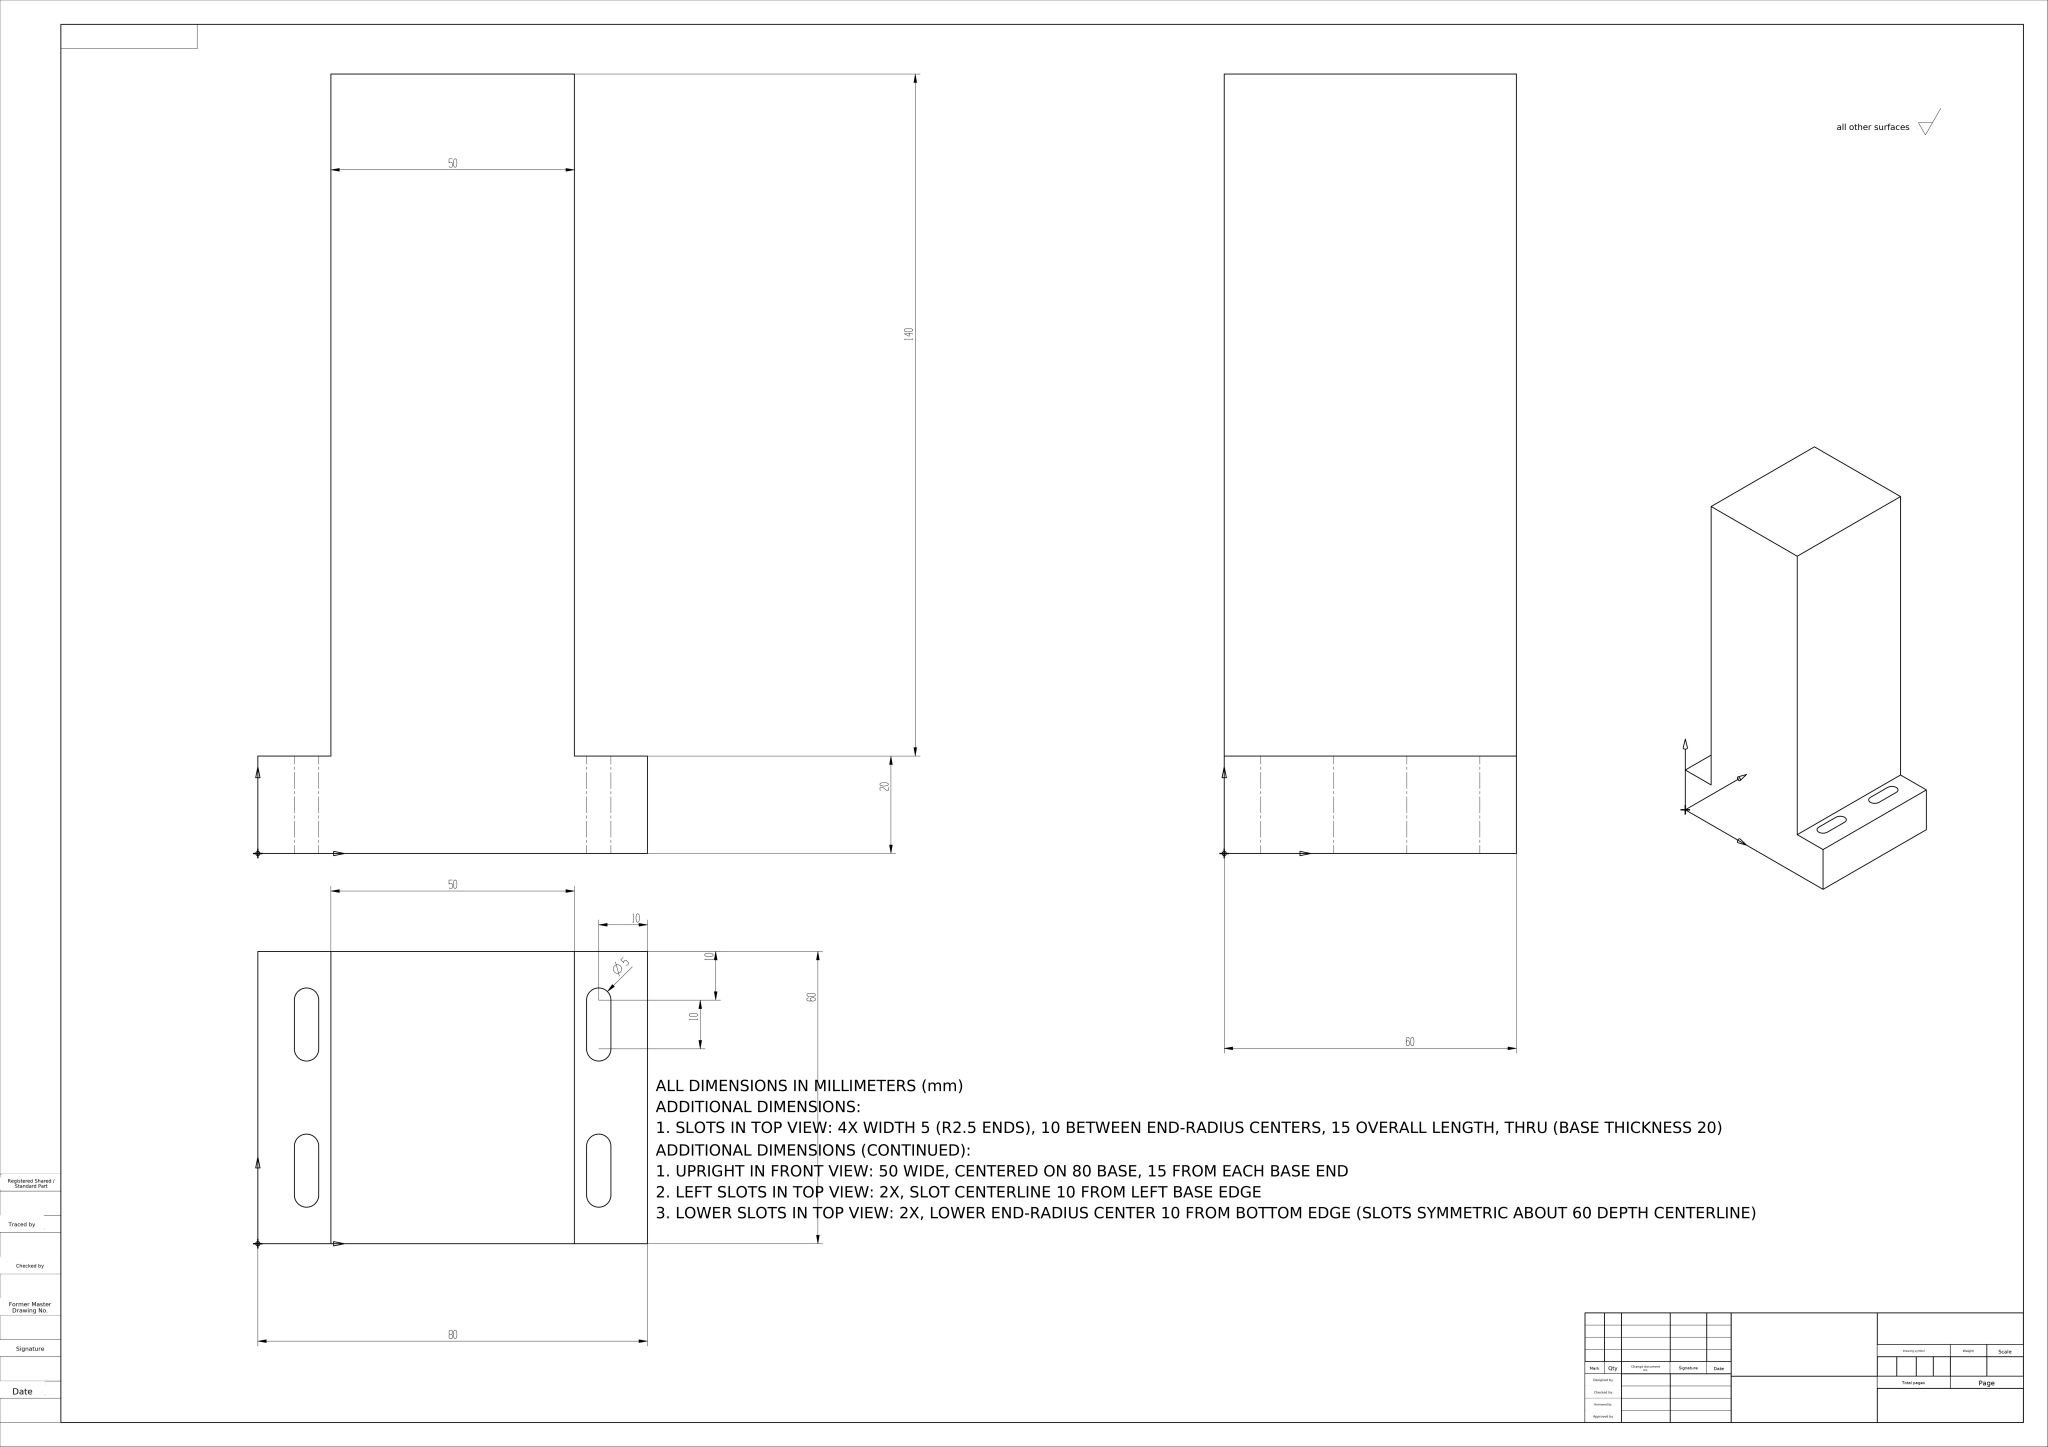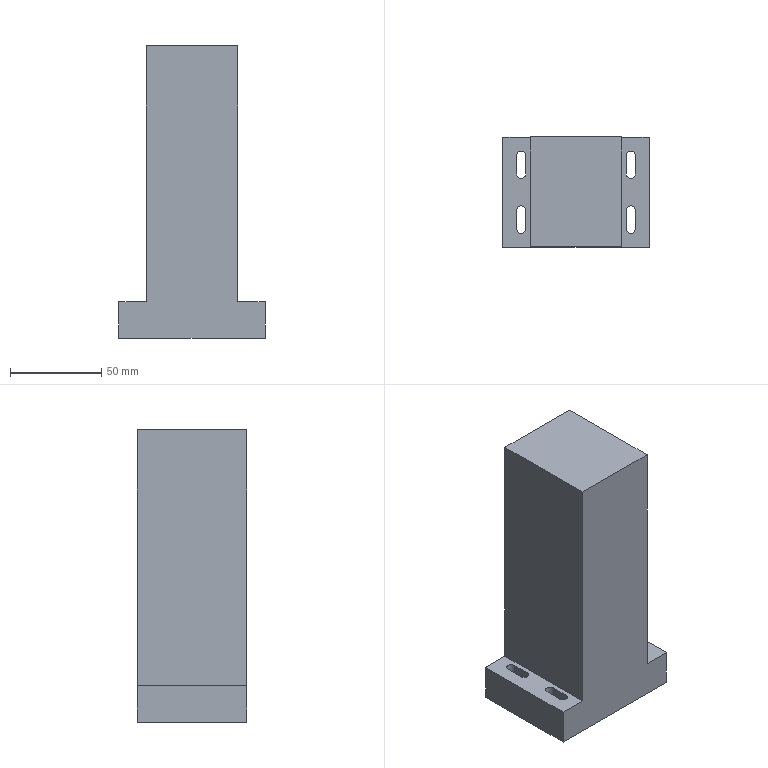Part | NX | mm | 1 solid | 26 faces | box 80 x 60 x 160 mm | volume 510429 mm3 | plane 18 | cylinder 8 | commonest cylinder face diameters 5 x8
STEP:
#1=CARTESIAN_POINT('',(0.,0.,0.));
#2=DIRECTION('',(0.,0.,1.));
#3=DIRECTION('',(1.,0.,0.));
#4=AXIS2_PLACEMENT_3D('',#1,#2,#3);
#5=(LENGTH_UNIT()NAMED_UNIT(*)SI_UNIT(.MILLI.,.METRE.));
#6=UNCERTAINTY_MEASURE_WITH_UNIT(LENGTH_MEASURE(0.00002),#5,'','');
#7=(NAMED_UNIT(*)PLANE_ANGLE_UNIT()SI_UNIT($,.RADIAN.));
#8=PLANE_ANGLE_MEASURE_WITH_UNIT(PLANE_ANGLE_MEASURE(0.01745),#7);
#9=DIMENSIONAL_EXPONENTS(0.,0.,0.,0.,0.,0.,0.);
#10=(CONVERSION_BASED_UNIT('',#8)NAMED_UNIT(#9)PLANE_ANGLE_UNIT());
#11=(NAMED_UNIT(*)SI_UNIT($,.STERADIAN.)SOLID_ANGLE_UNIT());
#12=(GEOMETRIC_REPRESENTATION_CONTEXT(3)GLOBAL_UNCERTAINTY_ASSIGNED_CONTEXT((#6))GLOBAL_UNIT_ASSIGNED_CONTEXT((#5,#10,#11))REPRESENTATION_CONTEXT('',''));
#13=SHAPE_REPRESENTATION('',(#4),#12);
#14=CARTESIAN_POINT('',(15.,60.,20.));
#15=VERTEX_POINT('',#14);
#16=CARTESIAN_POINT('',(15.,0.,20.));
#17=VERTEX_POINT('',#16);
#18=CARTESIAN_POINT('',(15.,60.,20.));
#19=DIRECTION('',(0.,-1.,0.));
#20=VECTOR('',#19,1.);
#21=LINE('',#18,#20);
#22=EDGE_CURVE('',#15,#17,#21,.T.);
#23=ORIENTED_EDGE('',*,*,#22,.T.);
#24=CARTESIAN_POINT('',(15.,-0.,160.));
#25=VERTEX_POINT('',#24);
#26=CARTESIAN_POINT('',(15.,-0.,160.));
#27=DIRECTION('',(0.,0.,-1.));
#28=VECTOR('',#27,1.);
#29=LINE('',#26,#28);
#30=EDGE_CURVE('',#25,#17,#29,.T.);
#31=ORIENTED_EDGE('',*,*,#30,.F.);
#32=CARTESIAN_POINT('',(15.,60.,160.));
#33=VERTEX_POINT('',#32);
#34=CARTESIAN_POINT('',(15.,60.,160.));
#35=DIRECTION('',(0.,-1.,0.));
#36=VECTOR('',#35,1.);
#37=LINE('',#34,#36);
#38=EDGE_CURVE('',#33,#25,#37,.T.);
#39=ORIENTED_EDGE('',*,*,#38,.F.);
#40=CARTESIAN_POINT('',(15.,60.,160.));
#41=DIRECTION('',(0.,0.,-1.));
#42=VECTOR('',#41,1.);
#43=LINE('',#40,#42);
#44=EDGE_CURVE('',#33,#15,#43,.T.);
#45=ORIENTED_EDGE('',*,*,#44,.T.);
#46=EDGE_LOOP('',(#23,#31,#39,#45));
#47=FACE_OUTER_BOUND('',#46,.T.);
#48=CARTESIAN_POINT('',(15.,60.,160.));
#49=DIRECTION('',(1.,0.,0.));
#50=DIRECTION('',(-0.,1.,0.));
#51=AXIS2_PLACEMENT_3D('',#48,#49,#50);
#52=PLANE('',#51);
#53=ADVANCED_FACE('',(#47),#52,.F.);
#54=ORIENTED_EDGE('',*,*,#30,.T.);
#55=CARTESIAN_POINT('',(0.,0.,20.));
#56=VERTEX_POINT('',#55);
#57=CARTESIAN_POINT('',(40.,0.,20.));
#58=DIRECTION('',(-1.,0.,0.));
#59=VECTOR('',#58,1.);
#60=LINE('',#57,#59);
#61=EDGE_CURVE('',#17,#56,#60,.T.);
#62=ORIENTED_EDGE('',*,*,#61,.T.);
#63=CARTESIAN_POINT('',(0.,0.,0.));
#64=VERTEX_POINT('',#63);
#65=CARTESIAN_POINT('',(0.,0.,0.));
#66=DIRECTION('',(0.,0.,1.));
#67=VECTOR('',#66,1.);
#68=LINE('',#65,#67);
#69=EDGE_CURVE('',#64,#56,#68,.T.);
#70=ORIENTED_EDGE('',*,*,#69,.F.);
#71=CARTESIAN_POINT('',(80.,0.,0.));
#72=VERTEX_POINT('',#71);
#73=CARTESIAN_POINT('',(40.,0.,0.));
#74=DIRECTION('',(1.,0.,0.));
#75=VECTOR('',#74,1.);
#76=LINE('',#73,#75);
#77=EDGE_CURVE('',#64,#72,#76,.T.);
#78=ORIENTED_EDGE('',*,*,#77,.T.);
#79=CARTESIAN_POINT('',(80.,0.,20.));
#80=VERTEX_POINT('',#79);
#81=CARTESIAN_POINT('',(80.,0.,0.));
#82=DIRECTION('',(0.,0.,1.));
#83=VECTOR('',#82,1.);
#84=LINE('',#81,#83);
#85=EDGE_CURVE('',#72,#80,#84,.T.);
#86=ORIENTED_EDGE('',*,*,#85,.T.);
#87=CARTESIAN_POINT('',(65.,0.,20.));
#88=VERTEX_POINT('',#87);
#89=CARTESIAN_POINT('',(40.,0.,20.));
#90=DIRECTION('',(-1.,0.,0.));
#91=VECTOR('',#90,1.);
#92=LINE('',#89,#91);
#93=EDGE_CURVE('',#80,#88,#92,.T.);
#94=ORIENTED_EDGE('',*,*,#93,.T.);
#95=CARTESIAN_POINT('',(65.,0.,160.));
#96=VERTEX_POINT('',#95);
#97=CARTESIAN_POINT('',(65.,0.,160.));
#98=DIRECTION('',(0.,0.,-1.));
#99=VECTOR('',#98,1.);
#100=LINE('',#97,#99);
#101=EDGE_CURVE('',#96,#88,#100,.T.);
#102=ORIENTED_EDGE('',*,*,#101,.F.);
#103=CARTESIAN_POINT('',(15.,-0.,160.));
#104=DIRECTION('',(1.,0.,0.));
#105=VECTOR('',#104,1.);
#106=LINE('',#103,#105);
#107=EDGE_CURVE('',#25,#96,#106,.T.);
#108=ORIENTED_EDGE('',*,*,#107,.F.);
#109=EDGE_LOOP('',(#54,#62,#70,#78,#86,#94,#102,#108));
#110=FACE_OUTER_BOUND('',#109,.T.);
#111=CARTESIAN_POINT('',(15.,-0.,160.));
#112=DIRECTION('',(-0.,1.,0.));
#113=DIRECTION('',(-1.,-0.,0.));
#114=AXIS2_PLACEMENT_3D('',#111,#112,#113);
#115=PLANE('',#114);
#116=ADVANCED_FACE('',(#110),#115,.F.);
#117=CARTESIAN_POINT('',(65.,60.,20.));
#118=VERTEX_POINT('',#117);
#119=CARTESIAN_POINT('',(65.,0.,20.));
#120=DIRECTION('',(0.,1.,0.));
#121=VECTOR('',#120,1.);
#122=LINE('',#119,#121);
#123=EDGE_CURVE('',#88,#118,#122,.T.);
#124=ORIENTED_EDGE('',*,*,#123,.T.);
#125=CARTESIAN_POINT('',(65.,60.,160.));
#126=VERTEX_POINT('',#125);
#127=CARTESIAN_POINT('',(65.,60.,160.));
#128=DIRECTION('',(0.,0.,-1.));
#129=VECTOR('',#128,1.);
#130=LINE('',#127,#129);
#131=EDGE_CURVE('',#126,#118,#130,.T.);
#132=ORIENTED_EDGE('',*,*,#131,.F.);
#133=CARTESIAN_POINT('',(65.,0.,160.));
#134=DIRECTION('',(0.,1.,0.));
#135=VECTOR('',#134,1.);
#136=LINE('',#133,#135);
#137=EDGE_CURVE('',#96,#126,#136,.T.);
#138=ORIENTED_EDGE('',*,*,#137,.F.);
#139=ORIENTED_EDGE('',*,*,#101,.T.);
#140=EDGE_LOOP('',(#124,#132,#138,#139));
#141=FACE_OUTER_BOUND('',#140,.T.);
#142=CARTESIAN_POINT('',(65.,0.,160.));
#143=DIRECTION('',(-1.,0.,0.));
#144=DIRECTION('',(0.,0.,1.));
#145=AXIS2_PLACEMENT_3D('',#142,#143,#144);
#146=PLANE('',#145);
#147=ADVANCED_FACE('',(#141),#146,.F.);
#148=ORIENTED_EDGE('',*,*,#131,.T.);
#149=CARTESIAN_POINT('',(80.,60.,20.));
#150=VERTEX_POINT('',#149);
#151=CARTESIAN_POINT('',(40.,60.,20.));
#152=DIRECTION('',(1.,0.,0.));
#153=VECTOR('',#152,1.);
#154=LINE('',#151,#153);
#155=EDGE_CURVE('',#118,#150,#154,.T.);
#156=ORIENTED_EDGE('',*,*,#155,.T.);
#157=CARTESIAN_POINT('',(80.,60.,0.));
#158=VERTEX_POINT('',#157);
#159=CARTESIAN_POINT('',(80.,60.,0.));
#160=DIRECTION('',(0.,0.,1.));
#161=VECTOR('',#160,1.);
#162=LINE('',#159,#161);
#163=EDGE_CURVE('',#158,#150,#162,.T.);
#164=ORIENTED_EDGE('',*,*,#163,.F.);
#165=CARTESIAN_POINT('',(0.,60.,0.));
#166=VERTEX_POINT('',#165);
#167=CARTESIAN_POINT('',(40.,60.,0.));
#168=DIRECTION('',(-1.,0.,0.));
#169=VECTOR('',#168,1.);
#170=LINE('',#167,#169);
#171=EDGE_CURVE('',#158,#166,#170,.T.);
#172=ORIENTED_EDGE('',*,*,#171,.T.);
#173=CARTESIAN_POINT('',(0.,60.,20.));
#174=VERTEX_POINT('',#173);
#175=CARTESIAN_POINT('',(0.,60.,0.));
#176=DIRECTION('',(0.,0.,1.));
#177=VECTOR('',#176,1.);
#178=LINE('',#175,#177);
#179=EDGE_CURVE('',#166,#174,#178,.T.);
#180=ORIENTED_EDGE('',*,*,#179,.T.);
#181=CARTESIAN_POINT('',(40.,60.,20.));
#182=DIRECTION('',(1.,0.,0.));
#183=VECTOR('',#182,1.);
#184=LINE('',#181,#183);
#185=EDGE_CURVE('',#174,#15,#184,.T.);
#186=ORIENTED_EDGE('',*,*,#185,.T.);
#187=ORIENTED_EDGE('',*,*,#44,.F.);
#188=CARTESIAN_POINT('',(65.,60.,160.));
#189=DIRECTION('',(-1.,-0.,0.));
#190=VECTOR('',#189,1.);
#191=LINE('',#188,#190);
#192=EDGE_CURVE('',#126,#33,#191,.T.);
#193=ORIENTED_EDGE('',*,*,#192,.F.);
#194=EDGE_LOOP('',(#148,#156,#164,#172,#180,#186,#187,#193));
#195=FACE_OUTER_BOUND('',#194,.T.);
#196=CARTESIAN_POINT('',(65.,60.,160.));
#197=DIRECTION('',(0.,-1.,0.));
#198=DIRECTION('',(1.,0.,0.));
#199=AXIS2_PLACEMENT_3D('',#196,#197,#198);
#200=PLANE('',#199);
#201=ADVANCED_FACE('',(#195),#200,.F.);
#202=ORIENTED_EDGE('',*,*,#38,.T.);
#203=ORIENTED_EDGE('',*,*,#107,.T.);
#204=ORIENTED_EDGE('',*,*,#137,.T.);
#205=ORIENTED_EDGE('',*,*,#192,.T.);
#206=EDGE_LOOP('',(#202,#203,#204,#205));
#207=FACE_OUTER_BOUND('',#206,.T.);
#208=CARTESIAN_POINT('',(0.,0.,160.));
#209=DIRECTION('',(0.,0.,1.));
#210=DIRECTION('',(1.,0.,0.));
#211=AXIS2_PLACEMENT_3D('',#208,#209,#210);
#212=PLANE('',#211);
#213=ADVANCED_FACE('',(#207),#212,.T.);
#214=CARTESIAN_POINT('',(7.5,20.,20.));
#215=VERTEX_POINT('',#214);
#216=CARTESIAN_POINT('',(7.5,10.,20.));
#217=VERTEX_POINT('',#216);
#218=CARTESIAN_POINT('',(7.5,20.,20.));
#219=DIRECTION('',(-0.,-1.,0.));
#220=VECTOR('',#219,1.);
#221=LINE('',#218,#220);
#222=EDGE_CURVE('',#215,#217,#221,.T.);
#223=ORIENTED_EDGE('',*,*,#222,.F.);
#224=CARTESIAN_POINT('',(12.5,20.,20.));
#225=VERTEX_POINT('',#224);
#226=CARTESIAN_POINT('',(10.,20.,20.));
#227=DIRECTION('',(0.,0.,1.));
#228=DIRECTION('',(0.,-1.,0.));
#229=AXIS2_PLACEMENT_3D('',#226,#227,#228);
#230=CIRCLE('',#229,2.5);
#231=EDGE_CURVE('',#225,#215,#230,.T.);
#232=ORIENTED_EDGE('',*,*,#231,.F.);
#233=CARTESIAN_POINT('',(12.5,10.,20.));
#234=VERTEX_POINT('',#233);
#235=CARTESIAN_POINT('',(12.5,10.,20.));
#236=DIRECTION('',(0.,1.,0.));
#237=VECTOR('',#236,1.);
#238=LINE('',#235,#237);
#239=EDGE_CURVE('',#234,#225,#238,.T.);
#240=ORIENTED_EDGE('',*,*,#239,.F.);
#241=CARTESIAN_POINT('',(10.,10.,20.));
#242=DIRECTION('',(0.,0.,1.));
#243=DIRECTION('',(0.,-1.,0.));
#244=AXIS2_PLACEMENT_3D('',#241,#242,#243);
#245=CIRCLE('',#244,2.5);
#246=EDGE_CURVE('',#217,#234,#245,.T.);
#247=ORIENTED_EDGE('',*,*,#246,.F.);
#248=EDGE_LOOP('',(#223,#232,#240,#247));
#249=FACE_BOUND('',#248,.T.);
#250=CARTESIAN_POINT('',(7.5,50.,20.));
#251=VERTEX_POINT('',#250);
#252=CARTESIAN_POINT('',(7.5,40.,20.));
#253=VERTEX_POINT('',#252);
#254=CARTESIAN_POINT('',(7.5,50.,20.));
#255=DIRECTION('',(0.,-1.,0.));
#256=VECTOR('',#255,1.);
#257=LINE('',#254,#256);
#258=EDGE_CURVE('',#251,#253,#257,.T.);
#259=ORIENTED_EDGE('',*,*,#258,.F.);
#260=CARTESIAN_POINT('',(12.5,50.,20.));
#261=VERTEX_POINT('',#260);
#262=CARTESIAN_POINT('',(10.,50.,20.));
#263=DIRECTION('',(0.,0.,1.));
#264=DIRECTION('',(0.,1.,0.));
#265=AXIS2_PLACEMENT_3D('',#262,#263,#264);
#266=CIRCLE('',#265,2.5);
#267=EDGE_CURVE('',#261,#251,#266,.T.);
#268=ORIENTED_EDGE('',*,*,#267,.F.);
#269=CARTESIAN_POINT('',(12.5,40.,20.));
#270=VERTEX_POINT('',#269);
#271=CARTESIAN_POINT('',(12.5,40.,20.));
#272=DIRECTION('',(0.,1.,0.));
#273=VECTOR('',#272,1.);
#274=LINE('',#271,#273);
#275=EDGE_CURVE('',#270,#261,#274,.T.);
#276=ORIENTED_EDGE('',*,*,#275,.F.);
#277=CARTESIAN_POINT('',(10.,40.,20.));
#278=DIRECTION('',(0.,0.,1.));
#279=DIRECTION('',(0.,1.,0.));
#280=AXIS2_PLACEMENT_3D('',#277,#278,#279);
#281=CIRCLE('',#280,2.5);
#282=EDGE_CURVE('',#253,#270,#281,.T.);
#283=ORIENTED_EDGE('',*,*,#282,.F.);
#284=EDGE_LOOP('',(#259,#268,#276,#283));
#285=FACE_BOUND('',#284,.T.);
#286=ORIENTED_EDGE('',*,*,#22,.F.);
#287=ORIENTED_EDGE('',*,*,#185,.F.);
#288=CARTESIAN_POINT('',(0.,30.,20.));
#289=DIRECTION('',(0.,1.,0.));
#290=VECTOR('',#289,1.);
#291=LINE('',#288,#290);
#292=EDGE_CURVE('',#56,#174,#291,.T.);
#293=ORIENTED_EDGE('',*,*,#292,.F.);
#294=ORIENTED_EDGE('',*,*,#61,.F.);
#295=EDGE_LOOP('',(#286,#287,#293,#294));
#296=FACE_BOUND('',#295,.T.);
#297=CARTESIAN_POINT('',(40.,30.,20.));
#298=DIRECTION('',(0.,0.,1.));
#299=DIRECTION('',(1.,0.,0.));
#300=AXIS2_PLACEMENT_3D('',#297,#298,#299);
#301=PLANE('',#300);
#302=ADVANCED_FACE('',(#249,#285,#296),#301,.T.);
#303=CARTESIAN_POINT('',(67.5,50.,20.));
#304=VERTEX_POINT('',#303);
#305=CARTESIAN_POINT('',(67.5,40.,20.));
#306=VERTEX_POINT('',#305);
#307=CARTESIAN_POINT('',(67.5,50.,20.));
#308=DIRECTION('',(0.,-1.,0.));
#309=VECTOR('',#308,1.);
#310=LINE('',#307,#309);
#311=EDGE_CURVE('',#304,#306,#310,.T.);
#312=ORIENTED_EDGE('',*,*,#311,.F.);
#313=CARTESIAN_POINT('',(72.5,50.,20.));
#314=VERTEX_POINT('',#313);
#315=CARTESIAN_POINT('',(70.,50.,20.));
#316=DIRECTION('',(0.,0.,1.));
#317=DIRECTION('',(0.,1.,0.));
#318=AXIS2_PLACEMENT_3D('',#315,#316,#317);
#319=CIRCLE('',#318,2.5);
#320=EDGE_CURVE('',#314,#304,#319,.T.);
#321=ORIENTED_EDGE('',*,*,#320,.F.);
#322=CARTESIAN_POINT('',(72.5,40.,20.));
#323=VERTEX_POINT('',#322);
#324=CARTESIAN_POINT('',(72.5,40.,20.));
#325=DIRECTION('',(0.,1.,0.));
#326=VECTOR('',#325,1.);
#327=LINE('',#324,#326);
#328=EDGE_CURVE('',#323,#314,#327,.T.);
#329=ORIENTED_EDGE('',*,*,#328,.F.);
#330=CARTESIAN_POINT('',(70.,40.,20.));
#331=DIRECTION('',(0.,0.,1.));
#332=DIRECTION('',(0.,1.,0.));
#333=AXIS2_PLACEMENT_3D('',#330,#331,#332);
#334=CIRCLE('',#333,2.5);
#335=EDGE_CURVE('',#306,#323,#334,.T.);
#336=ORIENTED_EDGE('',*,*,#335,.F.);
#337=EDGE_LOOP('',(#312,#321,#329,#336));
#338=FACE_BOUND('',#337,.T.);
#339=CARTESIAN_POINT('',(67.5,20.,20.));
#340=VERTEX_POINT('',#339);
#341=CARTESIAN_POINT('',(67.5,10.,20.));
#342=VERTEX_POINT('',#341);
#343=CARTESIAN_POINT('',(67.5,20.,20.));
#344=DIRECTION('',(-0.,-1.,0.));
#345=VECTOR('',#344,1.);
#346=LINE('',#343,#345);
#347=EDGE_CURVE('',#340,#342,#346,.T.);
#348=ORIENTED_EDGE('',*,*,#347,.F.);
#349=CARTESIAN_POINT('',(72.5,20.,20.));
#350=VERTEX_POINT('',#349);
#351=CARTESIAN_POINT('',(70.,20.,20.));
#352=DIRECTION('',(0.,0.,1.));
#353=DIRECTION('',(0.,-1.,0.));
#354=AXIS2_PLACEMENT_3D('',#351,#352,#353);
#355=CIRCLE('',#354,2.5);
#356=EDGE_CURVE('',#350,#340,#355,.T.);
#357=ORIENTED_EDGE('',*,*,#356,.F.);
#358=CARTESIAN_POINT('',(72.5,10.,20.));
#359=VERTEX_POINT('',#358);
#360=CARTESIAN_POINT('',(72.5,10.,20.));
#361=DIRECTION('',(0.,1.,0.));
#362=VECTOR('',#361,1.);
#363=LINE('',#360,#362);
#364=EDGE_CURVE('',#359,#350,#363,.T.);
#365=ORIENTED_EDGE('',*,*,#364,.F.);
#366=CARTESIAN_POINT('',(70.,10.,20.));
#367=DIRECTION('',(0.,0.,1.));
#368=DIRECTION('',(0.,-1.,0.));
#369=AXIS2_PLACEMENT_3D('',#366,#367,#368);
#370=CIRCLE('',#369,2.5);
#371=EDGE_CURVE('',#342,#359,#370,.T.);
#372=ORIENTED_EDGE('',*,*,#371,.F.);
#373=EDGE_LOOP('',(#348,#357,#365,#372));
#374=FACE_BOUND('',#373,.T.);
#375=ORIENTED_EDGE('',*,*,#123,.F.);
#376=ORIENTED_EDGE('',*,*,#93,.F.);
#377=CARTESIAN_POINT('',(80.,30.,20.));
#378=DIRECTION('',(0.,-1.,0.));
#379=VECTOR('',#378,1.);
#380=LINE('',#377,#379);
#381=EDGE_CURVE('',#150,#80,#380,.T.);
#382=ORIENTED_EDGE('',*,*,#381,.F.);
#383=ORIENTED_EDGE('',*,*,#155,.F.);
#384=EDGE_LOOP('',(#375,#376,#382,#383));
#385=FACE_BOUND('',#384,.T.);
#386=CARTESIAN_POINT('',(40.,30.,20.));
#387=DIRECTION('',(0.,0.,1.));
#388=DIRECTION('',(1.,0.,0.));
#389=AXIS2_PLACEMENT_3D('',#386,#387,#388);
#390=PLANE('',#389);
#391=ADVANCED_FACE('',(#338,#374,#385),#390,.T.);
#392=ORIENTED_EDGE('',*,*,#69,.T.);
#393=ORIENTED_EDGE('',*,*,#292,.T.);
#394=ORIENTED_EDGE('',*,*,#179,.F.);
#395=CARTESIAN_POINT('',(0.,30.,0.));
#396=DIRECTION('',(0.,-1.,0.));
#397=VECTOR('',#396,1.);
#398=LINE('',#395,#397);
#399=EDGE_CURVE('',#166,#64,#398,.T.);
#400=ORIENTED_EDGE('',*,*,#399,.T.);
#401=EDGE_LOOP('',(#392,#393,#394,#400));
#402=FACE_OUTER_BOUND('',#401,.T.);
#403=CARTESIAN_POINT('',(0.,30.,0.));
#404=DIRECTION('',(-1.,0.,0.));
#405=DIRECTION('',(0.,0.,1.));
#406=AXIS2_PLACEMENT_3D('',#403,#404,#405);
#407=PLANE('',#406);
#408=ADVANCED_FACE('',(#402),#407,.T.);
#409=CARTESIAN_POINT('',(67.5,10.,0.));
#410=VERTEX_POINT('',#409);
#411=CARTESIAN_POINT('',(67.5,20.,0.));
#412=VERTEX_POINT('',#411);
#413=CARTESIAN_POINT('',(67.5,30.,0.));
#414=DIRECTION('',(0.,1.,0.));
#415=VECTOR('',#414,1.);
#416=LINE('',#413,#415);
#417=EDGE_CURVE('',#410,#412,#416,.T.);
#418=ORIENTED_EDGE('',*,*,#417,.F.);
#419=CARTESIAN_POINT('',(72.5,10.,0.));
#420=VERTEX_POINT('',#419);
#421=CARTESIAN_POINT('',(70.,10.,0.));
#422=DIRECTION('',(0.,0.,-1.));
#423=DIRECTION('',(-1.,0.,0.));
#424=AXIS2_PLACEMENT_3D('',#421,#422,#423);
#425=CIRCLE('',#424,2.5);
#426=EDGE_CURVE('',#420,#410,#425,.T.);
#427=ORIENTED_EDGE('',*,*,#426,.F.);
#428=CARTESIAN_POINT('',(72.5,20.,0.));
#429=VERTEX_POINT('',#428);
#430=CARTESIAN_POINT('',(72.5,30.,0.));
#431=DIRECTION('',(-0.,-1.,0.));
#432=VECTOR('',#431,1.);
#433=LINE('',#430,#432);
#434=EDGE_CURVE('',#429,#420,#433,.T.);
#435=ORIENTED_EDGE('',*,*,#434,.F.);
#436=CARTESIAN_POINT('',(70.,20.,0.));
#437=DIRECTION('',(0.,0.,-1.));
#438=DIRECTION('',(-1.,0.,0.));
#439=AXIS2_PLACEMENT_3D('',#436,#437,#438);
#440=CIRCLE('',#439,2.5);
#441=EDGE_CURVE('',#412,#429,#440,.T.);
#442=ORIENTED_EDGE('',*,*,#441,.F.);
#443=EDGE_LOOP('',(#418,#427,#435,#442));
#444=FACE_BOUND('',#443,.T.);
#445=CARTESIAN_POINT('',(7.5,40.,0.));
#446=VERTEX_POINT('',#445);
#447=CARTESIAN_POINT('',(7.5,50.,0.));
#448=VERTEX_POINT('',#447);
#449=CARTESIAN_POINT('',(7.5,30.,0.));
#450=DIRECTION('',(0.,1.,0.));
#451=VECTOR('',#450,1.);
#452=LINE('',#449,#451);
#453=EDGE_CURVE('',#446,#448,#452,.T.);
#454=ORIENTED_EDGE('',*,*,#453,.F.);
#455=CARTESIAN_POINT('',(12.5,40.,0.));
#456=VERTEX_POINT('',#455);
#457=CARTESIAN_POINT('',(10.,40.,0.));
#458=DIRECTION('',(0.,0.,-1.));
#459=DIRECTION('',(-1.,0.,0.));
#460=AXIS2_PLACEMENT_3D('',#457,#458,#459);
#461=CIRCLE('',#460,2.5);
#462=EDGE_CURVE('',#456,#446,#461,.T.);
#463=ORIENTED_EDGE('',*,*,#462,.F.);
#464=CARTESIAN_POINT('',(12.5,50.,0.));
#465=VERTEX_POINT('',#464);
#466=CARTESIAN_POINT('',(12.5,30.,0.));
#467=DIRECTION('',(0.,-1.,0.));
#468=VECTOR('',#467,1.);
#469=LINE('',#466,#468);
#470=EDGE_CURVE('',#465,#456,#469,.T.);
#471=ORIENTED_EDGE('',*,*,#470,.F.);
#472=CARTESIAN_POINT('',(10.,50.,0.));
#473=DIRECTION('',(0.,0.,-1.));
#474=DIRECTION('',(-1.,0.,0.));
#475=AXIS2_PLACEMENT_3D('',#472,#473,#474);
#476=CIRCLE('',#475,2.5);
#477=EDGE_CURVE('',#448,#465,#476,.T.);
#478=ORIENTED_EDGE('',*,*,#477,.F.);
#479=EDGE_LOOP('',(#454,#463,#471,#478));
#480=FACE_BOUND('',#479,.T.);
#481=CARTESIAN_POINT('',(7.5,10.,0.));
#482=VERTEX_POINT('',#481);
#483=CARTESIAN_POINT('',(7.5,20.,0.));
#484=VERTEX_POINT('',#483);
#485=CARTESIAN_POINT('',(7.5,30.,0.));
#486=DIRECTION('',(0.,1.,0.));
#487=VECTOR('',#486,1.);
#488=LINE('',#485,#487);
#489=EDGE_CURVE('',#482,#484,#488,.T.);
#490=ORIENTED_EDGE('',*,*,#489,.F.);
#491=CARTESIAN_POINT('',(12.5,10.,0.));
#492=VERTEX_POINT('',#491);
#493=CARTESIAN_POINT('',(10.,10.,0.));
#494=DIRECTION('',(0.,0.,-1.));
#495=DIRECTION('',(-1.,0.,0.));
#496=AXIS2_PLACEMENT_3D('',#493,#494,#495);
#497=CIRCLE('',#496,2.5);
#498=EDGE_CURVE('',#492,#482,#497,.T.);
#499=ORIENTED_EDGE('',*,*,#498,.F.);
#500=CARTESIAN_POINT('',(12.5,20.,0.));
#501=VERTEX_POINT('',#500);
#502=CARTESIAN_POINT('',(12.5,30.,0.));
#503=DIRECTION('',(-0.,-1.,0.));
#504=VECTOR('',#503,1.);
#505=LINE('',#502,#504);
#506=EDGE_CURVE('',#501,#492,#505,.T.);
#507=ORIENTED_EDGE('',*,*,#506,.F.);
#508=CARTESIAN_POINT('',(10.,20.,0.));
#509=DIRECTION('',(0.,0.,-1.));
#510=DIRECTION('',(-1.,0.,0.));
#511=AXIS2_PLACEMENT_3D('',#508,#509,#510);
#512=CIRCLE('',#511,2.5);
#513=EDGE_CURVE('',#484,#501,#512,.T.);
#514=ORIENTED_EDGE('',*,*,#513,.F.);
#515=EDGE_LOOP('',(#490,#499,#507,#514));
#516=FACE_BOUND('',#515,.T.);
#517=CARTESIAN_POINT('',(67.5,40.,0.));
#518=VERTEX_POINT('',#517);
#519=CARTESIAN_POINT('',(67.5,50.,0.));
#520=VERTEX_POINT('',#519);
#521=CARTESIAN_POINT('',(67.5,30.,0.));
#522=DIRECTION('',(0.,1.,0.));
#523=VECTOR('',#522,1.);
#524=LINE('',#521,#523);
#525=EDGE_CURVE('',#518,#520,#524,.T.);
#526=ORIENTED_EDGE('',*,*,#525,.F.);
#527=CARTESIAN_POINT('',(72.5,40.,0.));
#528=VERTEX_POINT('',#527);
#529=CARTESIAN_POINT('',(70.,40.,0.));
#530=DIRECTION('',(0.,0.,-1.));
#531=DIRECTION('',(-1.,0.,0.));
#532=AXIS2_PLACEMENT_3D('',#529,#530,#531);
#533=CIRCLE('',#532,2.5);
#534=EDGE_CURVE('',#528,#518,#533,.T.);
#535=ORIENTED_EDGE('',*,*,#534,.F.);
#536=CARTESIAN_POINT('',(72.5,50.,0.));
#537=VERTEX_POINT('',#536);
#538=CARTESIAN_POINT('',(72.5,30.,0.));
#539=DIRECTION('',(0.,-1.,0.));
#540=VECTOR('',#539,1.);
#541=LINE('',#538,#540);
#542=EDGE_CURVE('',#537,#528,#541,.T.);
#543=ORIENTED_EDGE('',*,*,#542,.F.);
#544=CARTESIAN_POINT('',(70.,50.,0.));
#545=DIRECTION('',(0.,0.,-1.));
#546=DIRECTION('',(-1.,0.,0.));
#547=AXIS2_PLACEMENT_3D('',#544,#545,#546);
#548=CIRCLE('',#547,2.5);
#549=EDGE_CURVE('',#520,#537,#548,.T.);
#550=ORIENTED_EDGE('',*,*,#549,.F.);
#551=EDGE_LOOP('',(#526,#535,#543,#550));
#552=FACE_BOUND('',#551,.T.);
#553=CARTESIAN_POINT('',(80.,30.,0.));
#554=DIRECTION('',(0.,1.,0.));
#555=VECTOR('',#554,1.);
#556=LINE('',#553,#555);
#557=EDGE_CURVE('',#72,#158,#556,.T.);
#558=ORIENTED_EDGE('',*,*,#557,.F.);
#559=ORIENTED_EDGE('',*,*,#77,.F.);
#560=ORIENTED_EDGE('',*,*,#399,.F.);
#561=ORIENTED_EDGE('',*,*,#171,.F.);
#562=EDGE_LOOP('',(#558,#559,#560,#561));
#563=FACE_BOUND('',#562,.T.);
#564=CARTESIAN_POINT('',(40.,30.,0.));
#565=DIRECTION('',(0.,0.,-1.));
#566=DIRECTION('',(-1.,0.,0.));
#567=AXIS2_PLACEMENT_3D('',#564,#565,#566);
#568=PLANE('',#567);
#569=ADVANCED_FACE('',(#444,#480,#516,#552,#563),#568,.T.);
#570=ORIENTED_EDGE('',*,*,#557,.T.);
#571=ORIENTED_EDGE('',*,*,#163,.T.);
#572=ORIENTED_EDGE('',*,*,#381,.T.);
#573=ORIENTED_EDGE('',*,*,#85,.F.);
#574=EDGE_LOOP('',(#570,#571,#572,#573));
#575=FACE_OUTER_BOUND('',#574,.T.);
#576=CARTESIAN_POINT('',(80.,30.,0.));
#577=DIRECTION('',(1.,0.,0.));
#578=DIRECTION('',(0.,0.,-1.));
#579=AXIS2_PLACEMENT_3D('',#576,#577,#578);
#580=PLANE('',#579);
#581=ADVANCED_FACE('',(#575),#580,.T.);
#582=ORIENTED_EDGE('',*,*,#525,.T.);
#583=CARTESIAN_POINT('',(67.5,50.,-145.));
#584=DIRECTION('',(0.,0.,-1.));
#585=VECTOR('',#584,1.);
#586=LINE('',#583,#585);
#587=EDGE_CURVE('',#304,#520,#586,.T.);
#588=ORIENTED_EDGE('',*,*,#587,.F.);
#589=ORIENTED_EDGE('',*,*,#311,.T.);
#590=CARTESIAN_POINT('',(67.5,40.,-145.));
#591=DIRECTION('',(0.,0.,-1.));
#592=VECTOR('',#591,1.);
#593=LINE('',#590,#592);
#594=EDGE_CURVE('',#306,#518,#593,.T.);
#595=ORIENTED_EDGE('',*,*,#594,.T.);
#596=EDGE_LOOP('',(#582,#588,#589,#595));
#597=FACE_OUTER_BOUND('',#596,.T.);
#598=CARTESIAN_POINT('',(67.5,50.,-145.));
#599=DIRECTION('',(-1.,0.,0.));
#600=DIRECTION('',(0.,0.,1.));
#601=AXIS2_PLACEMENT_3D('',#598,#599,#600);
#602=PLANE('',#601);
#603=ADVANCED_FACE('',(#597),#602,.F.);
#604=ORIENTED_EDGE('',*,*,#534,.T.);
#605=ORIENTED_EDGE('',*,*,#594,.F.);
#606=ORIENTED_EDGE('',*,*,#335,.T.);
#607=CARTESIAN_POINT('',(72.5,40.,-145.));
#608=DIRECTION('',(0.,0.,-1.));
#609=VECTOR('',#608,1.);
#610=LINE('',#607,#609);
#611=EDGE_CURVE('',#323,#528,#610,.T.);
#612=ORIENTED_EDGE('',*,*,#611,.T.);
#613=EDGE_LOOP('',(#604,#605,#606,#612));
#614=FACE_OUTER_BOUND('',#613,.T.);
#615=CARTESIAN_POINT('',(70.,40.,-145.));
#616=DIRECTION('',(0.,0.,1.));
#617=DIRECTION('',(1.,0.,0.));
#618=AXIS2_PLACEMENT_3D('',#615,#616,#617);
#619=CYLINDRICAL_SURFACE('',#618,2.5);
#620=ADVANCED_FACE('',(#614),#619,.F.);
#621=ORIENTED_EDGE('',*,*,#542,.T.);
#622=ORIENTED_EDGE('',*,*,#611,.F.);
#623=ORIENTED_EDGE('',*,*,#328,.T.);
#624=CARTESIAN_POINT('',(72.5,50.,-145.));
#625=DIRECTION('',(0.,0.,-1.));
#626=VECTOR('',#625,1.);
#627=LINE('',#624,#626);
#628=EDGE_CURVE('',#314,#537,#627,.T.);
#629=ORIENTED_EDGE('',*,*,#628,.T.);
#630=EDGE_LOOP('',(#621,#622,#623,#629));
#631=FACE_OUTER_BOUND('',#630,.T.);
#632=CARTESIAN_POINT('',(72.5,40.,-145.));
#633=DIRECTION('',(1.,0.,0.));
#634=DIRECTION('',(0.,0.,-1.));
#635=AXIS2_PLACEMENT_3D('',#632,#633,#634);
#636=PLANE('',#635);
#637=ADVANCED_FACE('',(#631),#636,.F.);
#638=ORIENTED_EDGE('',*,*,#549,.T.);
#639=ORIENTED_EDGE('',*,*,#628,.F.);
#640=ORIENTED_EDGE('',*,*,#320,.T.);
#641=ORIENTED_EDGE('',*,*,#587,.T.);
#642=EDGE_LOOP('',(#638,#639,#640,#641));
#643=FACE_OUTER_BOUND('',#642,.T.);
#644=CARTESIAN_POINT('',(70.,50.,-145.));
#645=DIRECTION('',(0.,0.,1.));
#646=DIRECTION('',(1.,0.,0.));
#647=AXIS2_PLACEMENT_3D('',#644,#645,#646);
#648=CYLINDRICAL_SURFACE('',#647,2.5);
#649=ADVANCED_FACE('',(#643),#648,.F.);
#650=ORIENTED_EDGE('',*,*,#489,.T.);
#651=CARTESIAN_POINT('',(7.5,20.,-145.));
#652=DIRECTION('',(0.,0.,-1.));
#653=VECTOR('',#652,1.);
#654=LINE('',#651,#653);
#655=EDGE_CURVE('',#215,#484,#654,.T.);
#656=ORIENTED_EDGE('',*,*,#655,.F.);
#657=ORIENTED_EDGE('',*,*,#222,.T.);
#658=CARTESIAN_POINT('',(7.5,10.,-145.));
#659=DIRECTION('',(0.,0.,-1.));
#660=VECTOR('',#659,1.);
#661=LINE('',#658,#660);
#662=EDGE_CURVE('',#217,#482,#661,.T.);
#663=ORIENTED_EDGE('',*,*,#662,.T.);
#664=EDGE_LOOP('',(#650,#656,#657,#663));
#665=FACE_OUTER_BOUND('',#664,.T.);
#666=CARTESIAN_POINT('',(7.5,20.,-145.));
#667=DIRECTION('',(-1.,0.,0.));
#668=DIRECTION('',(-0.,-1.,0.));
#669=AXIS2_PLACEMENT_3D('',#666,#667,#668);
#670=PLANE('',#669);
#671=ADVANCED_FACE('',(#665),#670,.F.);
#672=ORIENTED_EDGE('',*,*,#498,.T.);
#673=ORIENTED_EDGE('',*,*,#662,.F.);
#674=ORIENTED_EDGE('',*,*,#246,.T.);
#675=CARTESIAN_POINT('',(12.5,10.,-145.));
#676=DIRECTION('',(0.,0.,-1.));
#677=VECTOR('',#676,1.);
#678=LINE('',#675,#677);
#679=EDGE_CURVE('',#234,#492,#678,.T.);
#680=ORIENTED_EDGE('',*,*,#679,.T.);
#681=EDGE_LOOP('',(#672,#673,#674,#680));
#682=FACE_OUTER_BOUND('',#681,.T.);
#683=CARTESIAN_POINT('',(10.,10.,-145.));
#684=DIRECTION('',(0.,0.,1.));
#685=DIRECTION('',(1.,0.,0.));
#686=AXIS2_PLACEMENT_3D('',#683,#684,#685);
#687=CYLINDRICAL_SURFACE('',#686,2.5);
#688=ADVANCED_FACE('',(#682),#687,.F.);
#689=ORIENTED_EDGE('',*,*,#506,.T.);
#690=ORIENTED_EDGE('',*,*,#679,.F.);
#691=ORIENTED_EDGE('',*,*,#239,.T.);
#692=CARTESIAN_POINT('',(12.5,20.,-145.));
#693=DIRECTION('',(0.,0.,-1.));
#694=VECTOR('',#693,1.);
#695=LINE('',#692,#694);
#696=EDGE_CURVE('',#225,#501,#695,.T.);
#697=ORIENTED_EDGE('',*,*,#696,.T.);
#698=EDGE_LOOP('',(#689,#690,#691,#697));
#699=FACE_OUTER_BOUND('',#698,.T.);
#700=CARTESIAN_POINT('',(12.5,10.,-145.));
#701=DIRECTION('',(1.,-0.,0.));
#702=DIRECTION('',(0.,1.,0.));
#703=AXIS2_PLACEMENT_3D('',#700,#701,#702);
#704=PLANE('',#703);
#705=ADVANCED_FACE('',(#699),#704,.F.);
#706=ORIENTED_EDGE('',*,*,#513,.T.);
#707=ORIENTED_EDGE('',*,*,#696,.F.);
#708=ORIENTED_EDGE('',*,*,#231,.T.);
#709=ORIENTED_EDGE('',*,*,#655,.T.);
#710=EDGE_LOOP('',(#706,#707,#708,#709));
#711=FACE_OUTER_BOUND('',#710,.T.);
#712=CARTESIAN_POINT('',(10.,20.,-145.));
#713=DIRECTION('',(0.,0.,1.));
#714=DIRECTION('',(1.,0.,0.));
#715=AXIS2_PLACEMENT_3D('',#712,#713,#714);
#716=CYLINDRICAL_SURFACE('',#715,2.5);
#717=ADVANCED_FACE('',(#711),#716,.F.);
#718=ORIENTED_EDGE('',*,*,#453,.T.);
#719=CARTESIAN_POINT('',(7.5,50.,-145.));
#720=DIRECTION('',(0.,0.,-1.));
#721=VECTOR('',#720,1.);
#722=LINE('',#719,#721);
#723=EDGE_CURVE('',#251,#448,#722,.T.);
#724=ORIENTED_EDGE('',*,*,#723,.F.);
#725=ORIENTED_EDGE('',*,*,#258,.T.);
#726=CARTESIAN_POINT('',(7.5,40.,-145.));
#727=DIRECTION('',(0.,0.,-1.));
#728=VECTOR('',#727,1.);
#729=LINE('',#726,#728);
#730=EDGE_CURVE('',#253,#446,#729,.T.);
#731=ORIENTED_EDGE('',*,*,#730,.T.);
#732=EDGE_LOOP('',(#718,#724,#725,#731));
#733=FACE_OUTER_BOUND('',#732,.T.);
#734=CARTESIAN_POINT('',(7.5,50.,-145.));
#735=DIRECTION('',(-1.,0.,0.));
#736=DIRECTION('',(0.,0.,1.));
#737=AXIS2_PLACEMENT_3D('',#734,#735,#736);
#738=PLANE('',#737);
#739=ADVANCED_FACE('',(#733),#738,.F.);
#740=ORIENTED_EDGE('',*,*,#462,.T.);
#741=ORIENTED_EDGE('',*,*,#730,.F.);
#742=ORIENTED_EDGE('',*,*,#282,.T.);
#743=CARTESIAN_POINT('',(12.5,40.,-145.));
#744=DIRECTION('',(0.,0.,-1.));
#745=VECTOR('',#744,1.);
#746=LINE('',#743,#745);
#747=EDGE_CURVE('',#270,#456,#746,.T.);
#748=ORIENTED_EDGE('',*,*,#747,.T.);
#749=EDGE_LOOP('',(#740,#741,#742,#748));
#750=FACE_OUTER_BOUND('',#749,.T.);
#751=CARTESIAN_POINT('',(10.,40.,-145.));
#752=DIRECTION('',(0.,0.,1.));
#753=DIRECTION('',(1.,0.,0.));
#754=AXIS2_PLACEMENT_3D('',#751,#752,#753);
#755=CYLINDRICAL_SURFACE('',#754,2.5);
#756=ADVANCED_FACE('',(#750),#755,.F.);
#757=ORIENTED_EDGE('',*,*,#470,.T.);
#758=ORIENTED_EDGE('',*,*,#747,.F.);
#759=ORIENTED_EDGE('',*,*,#275,.T.);
#760=CARTESIAN_POINT('',(12.5,50.,-145.));
#761=DIRECTION('',(0.,0.,-1.));
#762=VECTOR('',#761,1.);
#763=LINE('',#760,#762);
#764=EDGE_CURVE('',#261,#465,#763,.T.);
#765=ORIENTED_EDGE('',*,*,#764,.T.);
#766=EDGE_LOOP('',(#757,#758,#759,#765));
#767=FACE_OUTER_BOUND('',#766,.T.);
#768=CARTESIAN_POINT('',(12.5,40.,-145.));
#769=DIRECTION('',(1.,0.,0.));
#770=DIRECTION('',(0.,0.,-1.));
#771=AXIS2_PLACEMENT_3D('',#768,#769,#770);
#772=PLANE('',#771);
#773=ADVANCED_FACE('',(#767),#772,.F.);
#774=ORIENTED_EDGE('',*,*,#477,.T.);
#775=ORIENTED_EDGE('',*,*,#764,.F.);
#776=ORIENTED_EDGE('',*,*,#267,.T.);
#777=ORIENTED_EDGE('',*,*,#723,.T.);
#778=EDGE_LOOP('',(#774,#775,#776,#777));
#779=FACE_OUTER_BOUND('',#778,.T.);
#780=CARTESIAN_POINT('',(10.,50.,-145.));
#781=DIRECTION('',(0.,0.,1.));
#782=DIRECTION('',(1.,0.,0.));
#783=AXIS2_PLACEMENT_3D('',#780,#781,#782);
#784=CYLINDRICAL_SURFACE('',#783,2.5);
#785=ADVANCED_FACE('',(#779),#784,.F.);
#786=ORIENTED_EDGE('',*,*,#417,.T.);
#787=CARTESIAN_POINT('',(67.5,20.,-145.));
#788=DIRECTION('',(0.,0.,-1.));
#789=VECTOR('',#788,1.);
#790=LINE('',#787,#789);
#791=EDGE_CURVE('',#340,#412,#790,.T.);
#792=ORIENTED_EDGE('',*,*,#791,.F.);
#793=ORIENTED_EDGE('',*,*,#347,.T.);
#794=CARTESIAN_POINT('',(67.5,10.,-145.));
#795=DIRECTION('',(0.,0.,-1.));
#796=VECTOR('',#795,1.);
#797=LINE('',#794,#796);
#798=EDGE_CURVE('',#342,#410,#797,.T.);
#799=ORIENTED_EDGE('',*,*,#798,.T.);
#800=EDGE_LOOP('',(#786,#792,#793,#799));
#801=FACE_OUTER_BOUND('',#800,.T.);
#802=CARTESIAN_POINT('',(67.5,20.,-145.));
#803=DIRECTION('',(-1.,0.,0.));
#804=DIRECTION('',(-0.,-1.,0.));
#805=AXIS2_PLACEMENT_3D('',#802,#803,#804);
#806=PLANE('',#805);
#807=ADVANCED_FACE('',(#801),#806,.F.);
#808=ORIENTED_EDGE('',*,*,#426,.T.);
#809=ORIENTED_EDGE('',*,*,#798,.F.);
#810=ORIENTED_EDGE('',*,*,#371,.T.);
#811=CARTESIAN_POINT('',(72.5,10.,-145.));
#812=DIRECTION('',(0.,0.,-1.));
#813=VECTOR('',#812,1.);
#814=LINE('',#811,#813);
#815=EDGE_CURVE('',#359,#420,#814,.T.);
#816=ORIENTED_EDGE('',*,*,#815,.T.);
#817=EDGE_LOOP('',(#808,#809,#810,#816));
#818=FACE_OUTER_BOUND('',#817,.T.);
#819=CARTESIAN_POINT('',(70.,10.,-145.));
#820=DIRECTION('',(0.,0.,1.));
#821=DIRECTION('',(1.,0.,0.));
#822=AXIS2_PLACEMENT_3D('',#819,#820,#821);
#823=CYLINDRICAL_SURFACE('',#822,2.5);
#824=ADVANCED_FACE('',(#818),#823,.F.);
#825=ORIENTED_EDGE('',*,*,#434,.T.);
#826=ORIENTED_EDGE('',*,*,#815,.F.);
#827=ORIENTED_EDGE('',*,*,#364,.T.);
#828=CARTESIAN_POINT('',(72.5,20.,-145.));
#829=DIRECTION('',(0.,0.,-1.));
#830=VECTOR('',#829,1.);
#831=LINE('',#828,#830);
#832=EDGE_CURVE('',#350,#429,#831,.T.);
#833=ORIENTED_EDGE('',*,*,#832,.T.);
#834=EDGE_LOOP('',(#825,#826,#827,#833));
#835=FACE_OUTER_BOUND('',#834,.T.);
#836=CARTESIAN_POINT('',(72.5,10.,-145.));
#837=DIRECTION('',(1.,-0.,0.));
#838=DIRECTION('',(0.,1.,0.));
#839=AXIS2_PLACEMENT_3D('',#836,#837,#838);
#840=PLANE('',#839);
#841=ADVANCED_FACE('',(#835),#840,.F.);
#842=ORIENTED_EDGE('',*,*,#441,.T.);
#843=ORIENTED_EDGE('',*,*,#832,.F.);
#844=ORIENTED_EDGE('',*,*,#356,.T.);
#845=ORIENTED_EDGE('',*,*,#791,.T.);
#846=EDGE_LOOP('',(#842,#843,#844,#845));
#847=FACE_OUTER_BOUND('',#846,.T.);
#848=CARTESIAN_POINT('',(70.,20.,-145.));
#849=DIRECTION('',(0.,0.,1.));
#850=DIRECTION('',(1.,0.,0.));
#851=AXIS2_PLACEMENT_3D('',#848,#849,#850);
#852=CYLINDRICAL_SURFACE('',#851,2.5);
#853=ADVANCED_FACE('',(#847),#852,.F.);
#854=CLOSED_SHELL('',(#53,#116,#147,#201,#213,#302,#391,#408,#569,#581,#603,#620,#637,#649,#671,#688,#705,#717,#739,#756,#773,#785,#807,#824,#841,#853));
#855=MANIFOLD_SOLID_BREP('',#854);
#856=ADVANCED_BREP_SHAPE_REPRESENTATION('',(#855),#12);
#857=SHAPE_REPRESENTATION_RELATIONSHIP('','',#13,#856);
#858=PRESENTATION_LAYER_ASSIGNMENT('','',(#855));
#859=DRAUGHTING_PRE_DEFINED_COLOUR('');
#860=FILL_AREA_STYLE_COLOUR('',#859);
#861=FILL_AREA_STYLE('',(#860));
#862=SURFACE_STYLE_FILL_AREA(#861);
#863=SURFACE_SIDE_STYLE('',(#862));
#864=SURFACE_STYLE_USAGE(.BOTH.,#863);
#865=PRESENTATION_STYLE_ASSIGNMENT((#864));
#866=STYLED_ITEM('',(#865),#855);
#867=MECHANICAL_DESIGN_GEOMETRIC_PRESENTATION_REPRESENTATION('',(#866),#12);